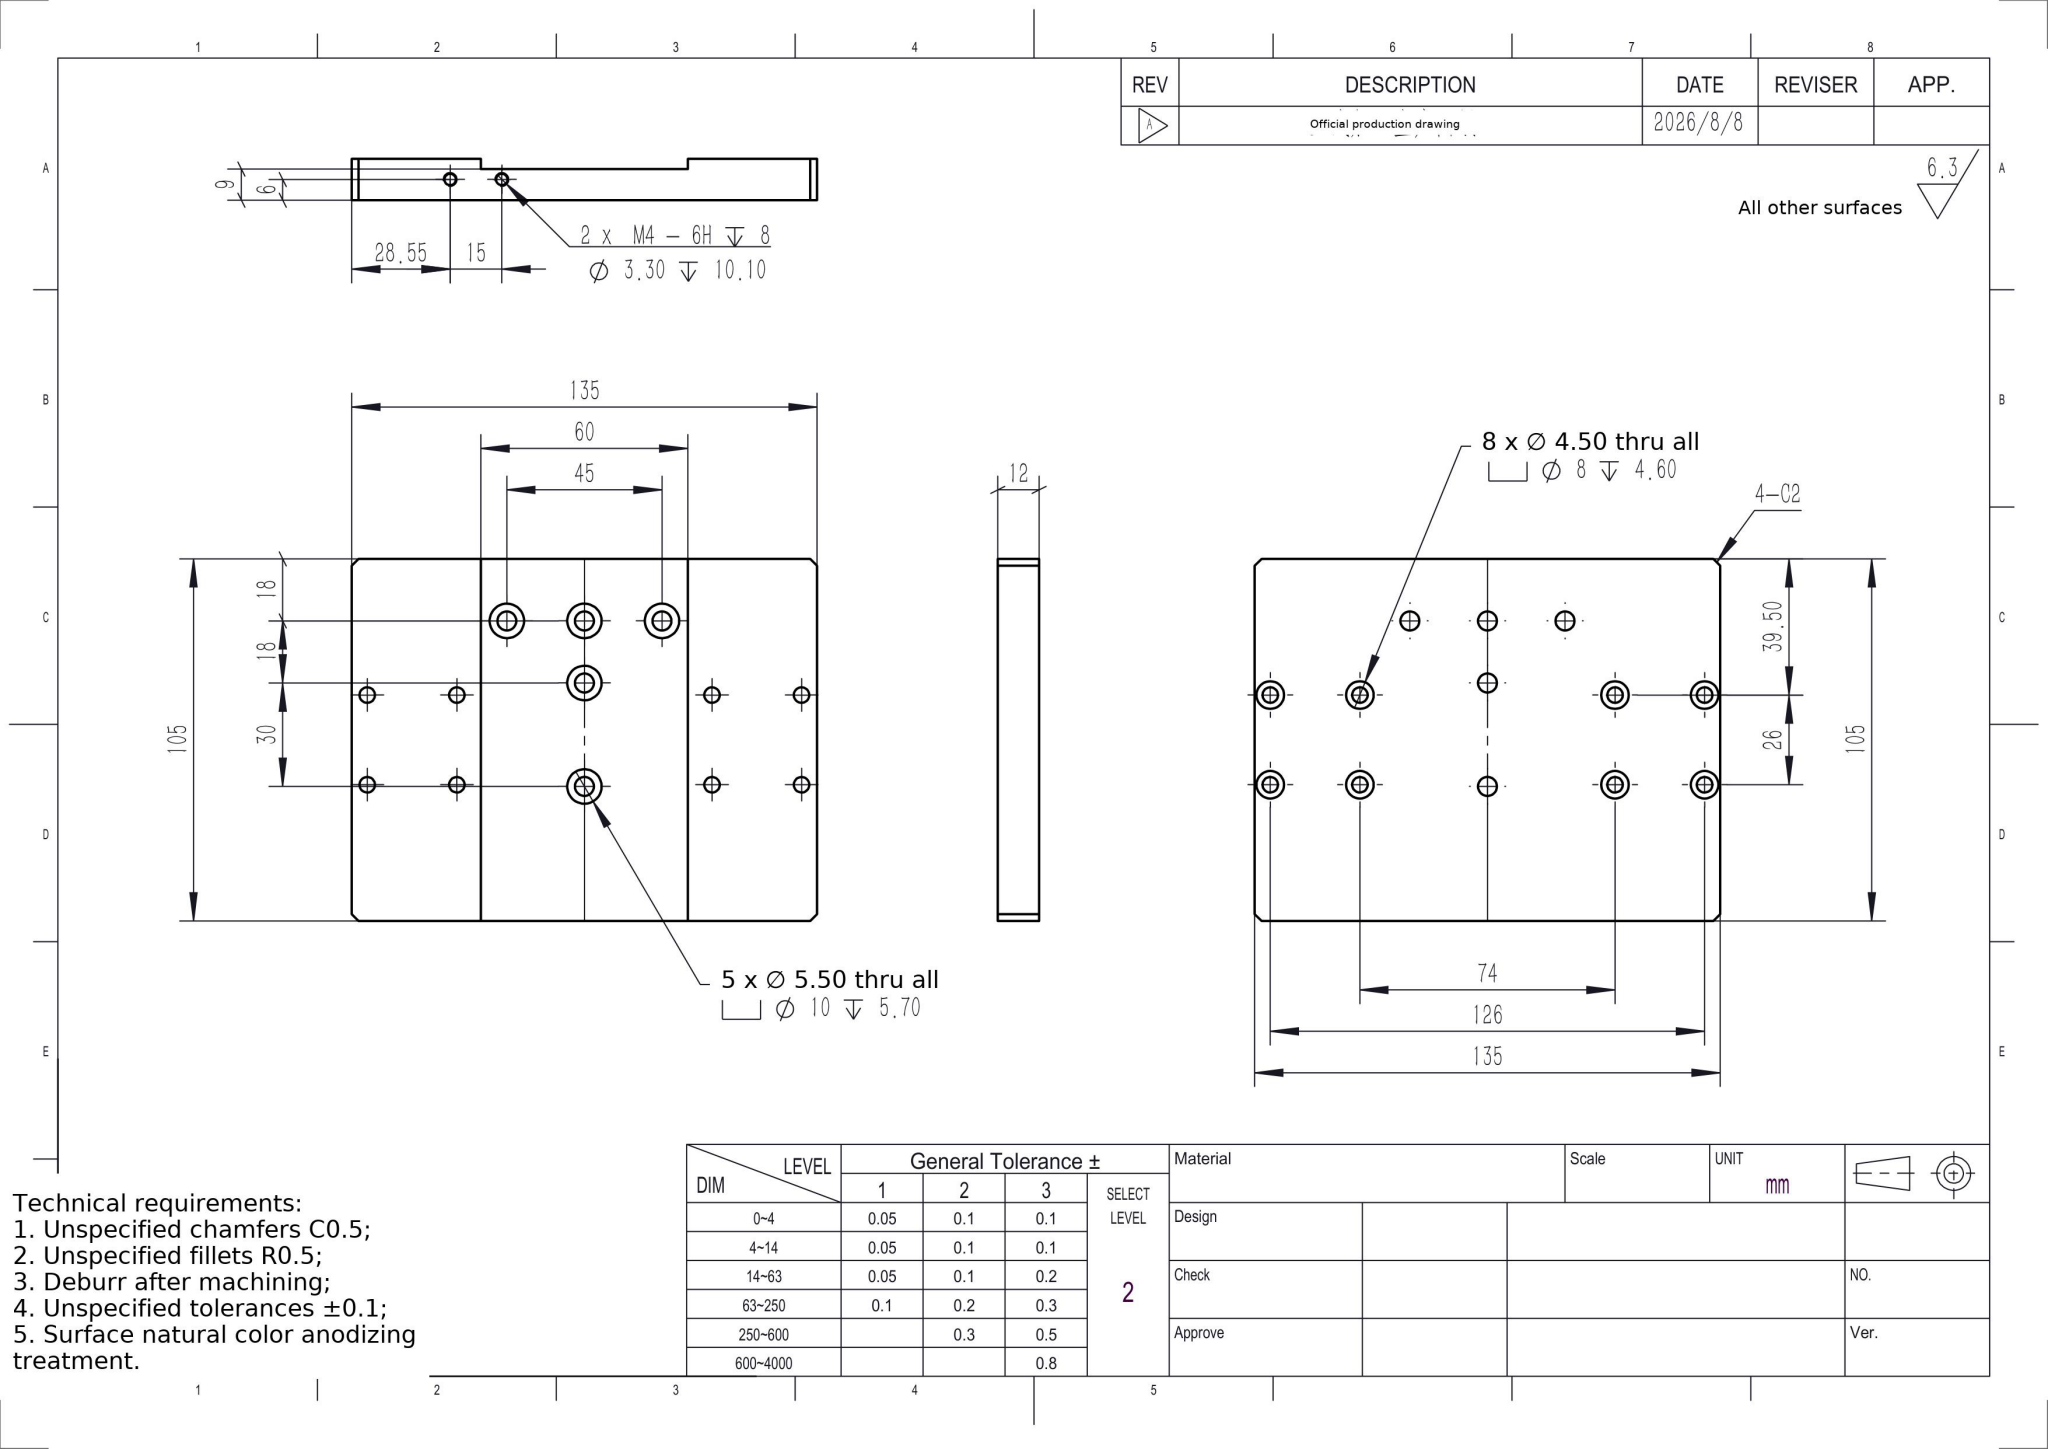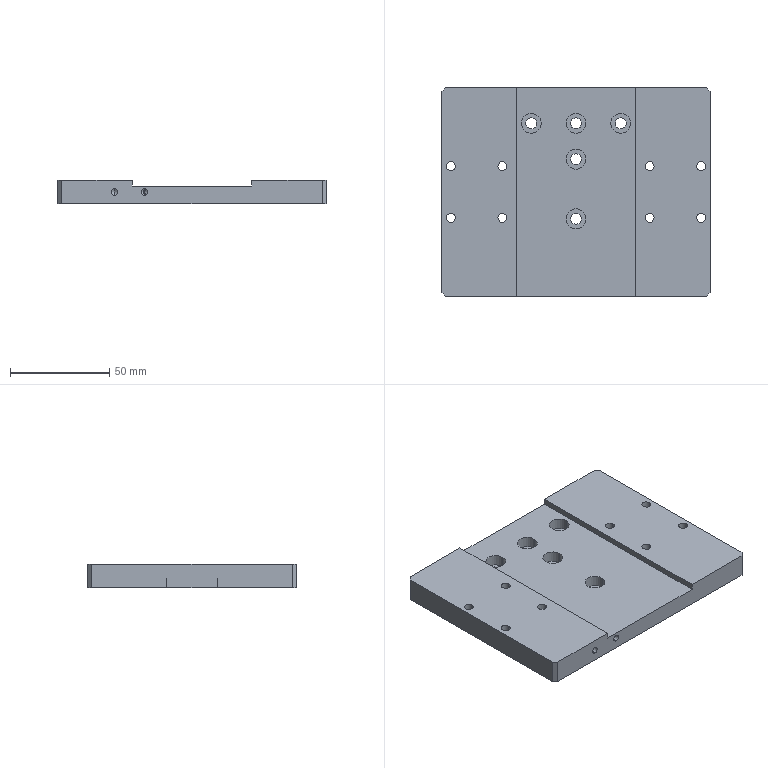Part | NX | mm | 1 solid | 87 faces | box 135 x 105 x 12 mm | volume 145504 mm3 | cylinder 56 | plane 27 | cone 4 | commonest cylinder face diameters 8 x16 4.5 x16 10 x10 5.5 x10 3.3 x4